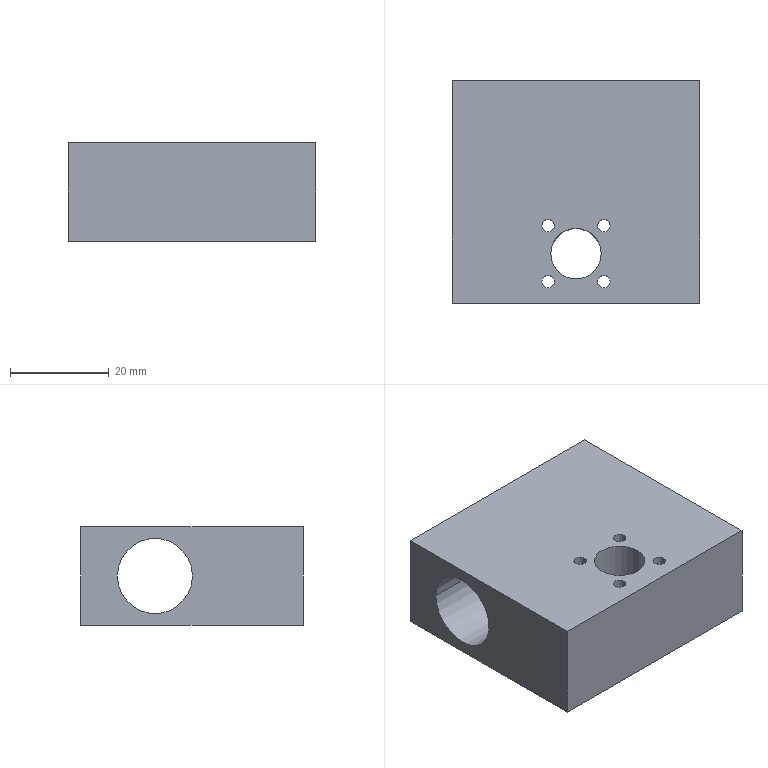Component | SolidWorks | Slider-1 | 1 solid | 18 faces | box 50 x 45 x 20 mm | volume 33900 mm3 | cylinder 12 | plane 6 | commonest cylinder face diameters 2.5 x8 15.2 x2 10.2 x2
STEP:
#1=CARTESIAN_POINT('',(0.9843,1.087,3.119));
#2=VERTEX_POINT('',#1);
#3=CARTESIAN_POINT('',(0.9843,0.4882,3.119));
#4=VERTEX_POINT('',#3);
#5=CARTESIAN_POINT('',(0.9843,0.7874,3.119));
#6=DIRECTION('',(-1.,-0.,0.));
#7=DIRECTION('',(-0.,1.,0.));
#8=AXIS2_PLACEMENT_3D('',#5,#6,#7);
#9=CIRCLE('',#8,0.2992);
#10=EDGE_CURVE('',#2,#4,#9,.T.);
#11=ORIENTED_EDGE('',*,*,#10,.F.);
#12=CARTESIAN_POINT('',(-0.9843,1.087,3.119));
#13=VERTEX_POINT('',#12);
#14=CARTESIAN_POINT('',(1.831,1.087,3.119));
#15=DIRECTION('',(-1.,-0.,0.));
#16=VECTOR('',#15,39.37);
#17=LINE('',#14,#16);
#18=EDGE_CURVE('',#2,#13,#17,.T.);
#19=ORIENTED_EDGE('',*,*,#18,.T.);
#20=CARTESIAN_POINT('',(-0.9843,0.4882,3.119));
#21=VERTEX_POINT('',#20);
#22=CARTESIAN_POINT('',(-0.9843,0.7874,3.119));
#23=DIRECTION('',(-1.,-0.,0.));
#24=DIRECTION('',(0.,-1.,0.));
#25=AXIS2_PLACEMENT_3D('',#22,#23,#24);
#26=CIRCLE('',#25,0.2992);
#27=EDGE_CURVE('',#13,#21,#26,.T.);
#28=ORIENTED_EDGE('',*,*,#27,.T.);
#29=CARTESIAN_POINT('',(1.831,0.4882,3.119));
#30=DIRECTION('',(-1.,-0.,0.));
#31=VECTOR('',#30,39.37);
#32=LINE('',#29,#31);
#33=EDGE_CURVE('',#4,#21,#32,.T.);
#34=ORIENTED_EDGE('',*,*,#33,.F.);
#35=EDGE_LOOP('',(#11,#19,#28,#34));
#36=FACE_OUTER_BOUND('',#35,.T.);
#37=CARTESIAN_POINT('',(1.831,0.7874,3.119));
#38=DIRECTION('',(-1.,-0.,0.));
#39=DIRECTION('',(0.,-1.,0.));
#40=AXIS2_PLACEMENT_3D('',#37,#38,#39);
#41=CYLINDRICAL_SURFACE('',#40,0.2992);
#42=ADVANCED_FACE('',(#36),#41,.F.);
#43=CARTESIAN_POINT('',(0.2719,-0.2227,2.725));
#44=VERTEX_POINT('',#43);
#45=CARTESIAN_POINT('',(0.1735,-0.2227,2.725));
#46=VERTEX_POINT('',#45);
#47=CARTESIAN_POINT('',(0.2227,-0.2227,2.725));
#48=DIRECTION('',(0.,0.,-1.));
#49=DIRECTION('',(1.,0.,0.));
#50=AXIS2_PLACEMENT_3D('',#47,#48,#49);
#51=CIRCLE('',#50,0.04921);
#52=EDGE_CURVE('',#44,#46,#51,.T.);
#53=ORIENTED_EDGE('',*,*,#52,.T.);
#54=CARTESIAN_POINT('',(0.1735,-0.2227,3.512));
#55=VERTEX_POINT('',#54);
#56=CARTESIAN_POINT('',(0.1735,-0.2227,2.586));
#57=DIRECTION('',(0.,0.,1.));
#58=VECTOR('',#57,39.37);
#59=LINE('',#56,#58);
#60=EDGE_CURVE('',#46,#55,#59,.T.);
#61=ORIENTED_EDGE('',*,*,#60,.T.);
#62=CARTESIAN_POINT('',(0.2719,-0.2227,3.512));
#63=VERTEX_POINT('',#62);
#64=CARTESIAN_POINT('',(0.2227,-0.2227,3.512));
#65=DIRECTION('',(0.,0.,1.));
#66=DIRECTION('',(1.,0.,0.));
#67=AXIS2_PLACEMENT_3D('',#64,#65,#66);
#68=CIRCLE('',#67,0.04921);
#69=EDGE_CURVE('',#55,#63,#68,.T.);
#70=ORIENTED_EDGE('',*,*,#69,.T.);
#71=CARTESIAN_POINT('',(0.2719,-0.2227,2.586));
#72=DIRECTION('',(0.,0.,1.));
#73=VECTOR('',#72,39.37);
#74=LINE('',#71,#73);
#75=EDGE_CURVE('',#44,#63,#74,.T.);
#76=ORIENTED_EDGE('',*,*,#75,.F.);
#77=EDGE_LOOP('',(#53,#61,#70,#76));
#78=FACE_OUTER_BOUND('',#77,.T.);
#79=CARTESIAN_POINT('',(0.2227,-0.2227,2.586));
#80=DIRECTION('',(0.,0.,1.));
#81=DIRECTION('',(1.,0.,0.));
#82=AXIS2_PLACEMENT_3D('',#79,#80,#81);
#83=CYLINDRICAL_SURFACE('',#82,0.04921);
#84=ADVANCED_FACE('',(#78),#83,.F.);
#85=CARTESIAN_POINT('',(-0.1735,-0.2227,2.725));
#86=VERTEX_POINT('',#85);
#87=CARTESIAN_POINT('',(-0.2719,-0.2227,2.725));
#88=VERTEX_POINT('',#87);
#89=CARTESIAN_POINT('',(-0.2227,-0.2227,2.725));
#90=DIRECTION('',(0.,0.,-1.));
#91=DIRECTION('',(1.,0.,0.));
#92=AXIS2_PLACEMENT_3D('',#89,#90,#91);
#93=CIRCLE('',#92,0.04921);
#94=EDGE_CURVE('',#86,#88,#93,.T.);
#95=ORIENTED_EDGE('',*,*,#94,.T.);
#96=CARTESIAN_POINT('',(-0.2719,-0.2227,3.512));
#97=VERTEX_POINT('',#96);
#98=CARTESIAN_POINT('',(-0.2719,-0.2227,2.586));
#99=DIRECTION('',(0.,0.,1.));
#100=VECTOR('',#99,39.37);
#101=LINE('',#98,#100);
#102=EDGE_CURVE('',#88,#97,#101,.T.);
#103=ORIENTED_EDGE('',*,*,#102,.T.);
#104=CARTESIAN_POINT('',(-0.1735,-0.2227,3.512));
#105=VERTEX_POINT('',#104);
#106=CARTESIAN_POINT('',(-0.2227,-0.2227,3.512));
#107=DIRECTION('',(0.,0.,1.));
#108=DIRECTION('',(1.,0.,0.));
#109=AXIS2_PLACEMENT_3D('',#106,#107,#108);
#110=CIRCLE('',#109,0.04921);
#111=EDGE_CURVE('',#97,#105,#110,.T.);
#112=ORIENTED_EDGE('',*,*,#111,.T.);
#113=CARTESIAN_POINT('',(-0.1735,-0.2227,2.586));
#114=DIRECTION('',(0.,0.,1.));
#115=VECTOR('',#114,39.37);
#116=LINE('',#113,#115);
#117=EDGE_CURVE('',#86,#105,#116,.T.);
#118=ORIENTED_EDGE('',*,*,#117,.F.);
#119=EDGE_LOOP('',(#95,#103,#112,#118));
#120=FACE_OUTER_BOUND('',#119,.T.);
#121=CARTESIAN_POINT('',(-0.2227,-0.2227,2.586));
#122=DIRECTION('',(0.,0.,1.));
#123=DIRECTION('',(1.,0.,0.));
#124=AXIS2_PLACEMENT_3D('',#121,#122,#123);
#125=CYLINDRICAL_SURFACE('',#124,0.04921);
#126=ADVANCED_FACE('',(#120),#125,.F.);
#127=CARTESIAN_POINT('',(0.2719,0.2227,2.725));
#128=VERTEX_POINT('',#127);
#129=CARTESIAN_POINT('',(0.1735,0.2227,2.725));
#130=VERTEX_POINT('',#129);
#131=CARTESIAN_POINT('',(0.2227,0.2227,2.725));
#132=DIRECTION('',(0.,0.,-1.));
#133=DIRECTION('',(1.,0.,0.));
#134=AXIS2_PLACEMENT_3D('',#131,#132,#133);
#135=CIRCLE('',#134,0.04921);
#136=EDGE_CURVE('',#128,#130,#135,.T.);
#137=ORIENTED_EDGE('',*,*,#136,.T.);
#138=CARTESIAN_POINT('',(0.1735,0.2227,3.512));
#139=VERTEX_POINT('',#138);
#140=CARTESIAN_POINT('',(0.1735,0.2227,2.586));
#141=DIRECTION('',(0.,0.,1.));
#142=VECTOR('',#141,39.37);
#143=LINE('',#140,#142);
#144=EDGE_CURVE('',#130,#139,#143,.T.);
#145=ORIENTED_EDGE('',*,*,#144,.T.);
#146=CARTESIAN_POINT('',(0.2719,0.2227,3.512));
#147=VERTEX_POINT('',#146);
#148=CARTESIAN_POINT('',(0.2227,0.2227,3.512));
#149=DIRECTION('',(0.,0.,1.));
#150=DIRECTION('',(1.,0.,0.));
#151=AXIS2_PLACEMENT_3D('',#148,#149,#150);
#152=CIRCLE('',#151,0.04921);
#153=EDGE_CURVE('',#139,#147,#152,.T.);
#154=ORIENTED_EDGE('',*,*,#153,.T.);
#155=CARTESIAN_POINT('',(0.2719,0.2227,2.586));
#156=DIRECTION('',(0.,0.,1.));
#157=VECTOR('',#156,39.37);
#158=LINE('',#155,#157);
#159=EDGE_CURVE('',#128,#147,#158,.T.);
#160=ORIENTED_EDGE('',*,*,#159,.F.);
#161=EDGE_LOOP('',(#137,#145,#154,#160));
#162=FACE_OUTER_BOUND('',#161,.T.);
#163=CARTESIAN_POINT('',(0.2227,0.2227,2.586));
#164=DIRECTION('',(0.,0.,1.));
#165=DIRECTION('',(1.,0.,0.));
#166=AXIS2_PLACEMENT_3D('',#163,#164,#165);
#167=CYLINDRICAL_SURFACE('',#166,0.04921);
#168=ADVANCED_FACE('',(#162),#167,.F.);
#169=CARTESIAN_POINT('',(-0.1735,0.2227,2.725));
#170=VERTEX_POINT('',#169);
#171=CARTESIAN_POINT('',(-0.2719,0.2227,2.725));
#172=VERTEX_POINT('',#171);
#173=CARTESIAN_POINT('',(-0.2227,0.2227,2.725));
#174=DIRECTION('',(0.,0.,-1.));
#175=DIRECTION('',(1.,0.,0.));
#176=AXIS2_PLACEMENT_3D('',#173,#174,#175);
#177=CIRCLE('',#176,0.04921);
#178=EDGE_CURVE('',#170,#172,#177,.T.);
#179=ORIENTED_EDGE('',*,*,#178,.T.);
#180=CARTESIAN_POINT('',(-0.2719,0.2227,3.512));
#181=VERTEX_POINT('',#180);
#182=CARTESIAN_POINT('',(-0.2719,0.2227,2.586));
#183=DIRECTION('',(0.,0.,1.));
#184=VECTOR('',#183,39.37);
#185=LINE('',#182,#184);
#186=EDGE_CURVE('',#172,#181,#185,.T.);
#187=ORIENTED_EDGE('',*,*,#186,.T.);
#188=CARTESIAN_POINT('',(-0.1735,0.2227,3.512));
#189=VERTEX_POINT('',#188);
#190=CARTESIAN_POINT('',(-0.2227,0.2227,3.512));
#191=DIRECTION('',(0.,0.,1.));
#192=DIRECTION('',(1.,0.,0.));
#193=AXIS2_PLACEMENT_3D('',#190,#191,#192);
#194=CIRCLE('',#193,0.04921);
#195=EDGE_CURVE('',#181,#189,#194,.T.);
#196=ORIENTED_EDGE('',*,*,#195,.T.);
#197=CARTESIAN_POINT('',(-0.1735,0.2227,2.586));
#198=DIRECTION('',(0.,0.,1.));
#199=VECTOR('',#198,39.37);
#200=LINE('',#197,#199);
#201=EDGE_CURVE('',#170,#189,#200,.T.);
#202=ORIENTED_EDGE('',*,*,#201,.F.);
#203=EDGE_LOOP('',(#179,#187,#196,#202));
#204=FACE_OUTER_BOUND('',#203,.T.);
#205=CARTESIAN_POINT('',(-0.2227,0.2227,2.586));
#206=DIRECTION('',(0.,0.,1.));
#207=DIRECTION('',(1.,0.,0.));
#208=AXIS2_PLACEMENT_3D('',#205,#206,#207);
#209=CYLINDRICAL_SURFACE('',#208,0.04921);
#210=ADVANCED_FACE('',(#204),#209,.F.);
#211=CARTESIAN_POINT('',(0.2008,0.,2.725));
#212=VERTEX_POINT('',#211);
#213=CARTESIAN_POINT('',(-0.2008,0.,2.725));
#214=VERTEX_POINT('',#213);
#215=CARTESIAN_POINT('',(-0.,0.,2.725));
#216=DIRECTION('',(0.,0.,-1.));
#217=DIRECTION('',(1.,0.,0.));
#218=AXIS2_PLACEMENT_3D('',#215,#216,#217);
#219=CIRCLE('',#218,0.2008);
#220=EDGE_CURVE('',#212,#214,#219,.T.);
#221=ORIENTED_EDGE('',*,*,#220,.T.);
#222=CARTESIAN_POINT('',(-0.2008,0.,3.512));
#223=VERTEX_POINT('',#222);
#224=CARTESIAN_POINT('',(-0.2008,0.,2.157));
#225=DIRECTION('',(0.,0.,1.));
#226=VECTOR('',#225,39.37);
#227=LINE('',#224,#226);
#228=EDGE_CURVE('',#214,#223,#227,.T.);
#229=ORIENTED_EDGE('',*,*,#228,.T.);
#230=CARTESIAN_POINT('',(0.2008,0.,3.512));
#231=VERTEX_POINT('',#230);
#232=CARTESIAN_POINT('',(-0.,0.,3.512));
#233=DIRECTION('',(0.,0.,1.));
#234=DIRECTION('',(1.,0.,0.));
#235=AXIS2_PLACEMENT_3D('',#232,#233,#234);
#236=CIRCLE('',#235,0.2008);
#237=EDGE_CURVE('',#223,#231,#236,.T.);
#238=ORIENTED_EDGE('',*,*,#237,.T.);
#239=CARTESIAN_POINT('',(0.2008,0.,2.157));
#240=DIRECTION('',(0.,0.,1.));
#241=VECTOR('',#240,39.37);
#242=LINE('',#239,#241);
#243=EDGE_CURVE('',#212,#231,#242,.T.);
#244=ORIENTED_EDGE('',*,*,#243,.F.);
#245=EDGE_LOOP('',(#221,#229,#238,#244));
#246=FACE_OUTER_BOUND('',#245,.T.);
#247=CARTESIAN_POINT('',(-0.,0.,2.157));
#248=DIRECTION('',(0.,0.,1.));
#249=DIRECTION('',(1.,0.,0.));
#250=AXIS2_PLACEMENT_3D('',#247,#248,#249);
#251=CYLINDRICAL_SURFACE('',#250,0.2008);
#252=ADVANCED_FACE('',(#246),#251,.F.);
#253=CARTESIAN_POINT('',(-0.9843,0.7874,3.119));
#254=DIRECTION('',(-1.,-0.,0.));
#255=DIRECTION('',(0.,-1.,0.));
#256=AXIS2_PLACEMENT_3D('',#253,#254,#255);
#257=CIRCLE('',#256,0.2992);
#258=EDGE_CURVE('',#21,#13,#257,.T.);
#259=ORIENTED_EDGE('',*,*,#258,.F.);
#260=ORIENTED_EDGE('',*,*,#27,.F.);
#261=EDGE_LOOP('',(#259,#260));
#262=FACE_BOUND('',#261,.T.);
#263=CARTESIAN_POINT('',(-0.9843,1.378,3.512));
#264=VERTEX_POINT('',#263);
#265=CARTESIAN_POINT('',(-0.9843,-0.3937,3.512));
#266=VERTEX_POINT('',#265);
#267=CARTESIAN_POINT('',(-0.9843,1.378,3.512));
#268=DIRECTION('',(0.,-1.,0.));
#269=VECTOR('',#268,39.37);
#270=LINE('',#267,#269);
#271=EDGE_CURVE('',#264,#266,#270,.T.);
#272=ORIENTED_EDGE('',*,*,#271,.F.);
#273=CARTESIAN_POINT('',(-0.9843,1.378,2.725));
#274=VERTEX_POINT('',#273);
#275=CARTESIAN_POINT('',(-0.9843,1.378,2.725));
#276=DIRECTION('',(0.,0.,1.));
#277=VECTOR('',#276,39.37);
#278=LINE('',#275,#277);
#279=EDGE_CURVE('',#274,#264,#278,.T.);
#280=ORIENTED_EDGE('',*,*,#279,.F.);
#281=CARTESIAN_POINT('',(-0.9843,-0.3937,2.725));
#282=VERTEX_POINT('',#281);
#283=CARTESIAN_POINT('',(-0.9843,1.378,2.725));
#284=DIRECTION('',(0.,-1.,0.));
#285=VECTOR('',#284,39.37);
#286=LINE('',#283,#285);
#287=EDGE_CURVE('',#274,#282,#286,.T.);
#288=ORIENTED_EDGE('',*,*,#287,.T.);
#289=CARTESIAN_POINT('',(-0.9843,-0.3937,2.725));
#290=DIRECTION('',(0.,0.,1.));
#291=VECTOR('',#290,39.37);
#292=LINE('',#289,#291);
#293=EDGE_CURVE('',#282,#266,#292,.T.);
#294=ORIENTED_EDGE('',*,*,#293,.T.);
#295=EDGE_LOOP('',(#272,#280,#288,#294));
#296=FACE_OUTER_BOUND('',#295,.T.);
#297=CARTESIAN_POINT('',(-0.9843,1.378,2.725));
#298=DIRECTION('',(-1.,-0.,0.));
#299=DIRECTION('',(0.,-1.,0.));
#300=AXIS2_PLACEMENT_3D('',#297,#298,#299);
#301=PLANE('',#300);
#302=ADVANCED_FACE('',(#262,#296),#301,.T.);
#303=CARTESIAN_POINT('',(0.9843,1.378,3.512));
#304=VERTEX_POINT('',#303);
#305=CARTESIAN_POINT('',(-0.9843,1.378,3.512));
#306=DIRECTION('',(-1.,-0.,0.));
#307=VECTOR('',#306,39.37);
#308=LINE('',#305,#307);
#309=EDGE_CURVE('',#304,#264,#308,.T.);
#310=ORIENTED_EDGE('',*,*,#309,.F.);
#311=CARTESIAN_POINT('',(0.9843,1.378,2.725));
#312=VERTEX_POINT('',#311);
#313=CARTESIAN_POINT('',(0.9843,1.378,2.725));
#314=DIRECTION('',(0.,0.,1.));
#315=VECTOR('',#314,39.37);
#316=LINE('',#313,#315);
#317=EDGE_CURVE('',#312,#304,#316,.T.);
#318=ORIENTED_EDGE('',*,*,#317,.F.);
#319=CARTESIAN_POINT('',(-0.9843,1.378,2.725));
#320=DIRECTION('',(-1.,-0.,0.));
#321=VECTOR('',#320,39.37);
#322=LINE('',#319,#321);
#323=EDGE_CURVE('',#312,#274,#322,.T.);
#324=ORIENTED_EDGE('',*,*,#323,.T.);
#325=ORIENTED_EDGE('',*,*,#279,.T.);
#326=EDGE_LOOP('',(#310,#318,#324,#325));
#327=FACE_OUTER_BOUND('',#326,.T.);
#328=CARTESIAN_POINT('',(-0.9843,1.378,2.725));
#329=DIRECTION('',(-0.,1.,0.));
#330=DIRECTION('',(-1.,-0.,0.));
#331=AXIS2_PLACEMENT_3D('',#328,#329,#330);
#332=PLANE('',#331);
#333=ADVANCED_FACE('',(#327),#332,.T.);
#334=CARTESIAN_POINT('',(0.9843,0.7874,3.119));
#335=DIRECTION('',(-1.,-0.,0.));
#336=DIRECTION('',(-0.,1.,0.));
#337=AXIS2_PLACEMENT_3D('',#334,#335,#336);
#338=CIRCLE('',#337,0.2992);
#339=EDGE_CURVE('',#4,#2,#338,.T.);
#340=ORIENTED_EDGE('',*,*,#339,.T.);
#341=ORIENTED_EDGE('',*,*,#10,.T.);
#342=EDGE_LOOP('',(#340,#341));
#343=FACE_BOUND('',#342,.T.);
#344=CARTESIAN_POINT('',(0.9843,-0.3937,3.512));
#345=VERTEX_POINT('',#344);
#346=CARTESIAN_POINT('',(0.9843,1.378,3.512));
#347=DIRECTION('',(-0.,1.,0.));
#348=VECTOR('',#347,39.37);
#349=LINE('',#346,#348);
#350=EDGE_CURVE('',#345,#304,#349,.T.);
#351=ORIENTED_EDGE('',*,*,#350,.F.);
#352=CARTESIAN_POINT('',(0.9843,-0.3937,2.725));
#353=VERTEX_POINT('',#352);
#354=CARTESIAN_POINT('',(0.9843,-0.3937,2.725));
#355=DIRECTION('',(0.,0.,1.));
#356=VECTOR('',#355,39.37);
#357=LINE('',#354,#356);
#358=EDGE_CURVE('',#353,#345,#357,.T.);
#359=ORIENTED_EDGE('',*,*,#358,.F.);
#360=CARTESIAN_POINT('',(0.9843,1.378,2.725));
#361=DIRECTION('',(-0.,1.,0.));
#362=VECTOR('',#361,39.37);
#363=LINE('',#360,#362);
#364=EDGE_CURVE('',#353,#312,#363,.T.);
#365=ORIENTED_EDGE('',*,*,#364,.T.);
#366=ORIENTED_EDGE('',*,*,#317,.T.);
#367=EDGE_LOOP('',(#351,#359,#365,#366));
#368=FACE_OUTER_BOUND('',#367,.T.);
#369=CARTESIAN_POINT('',(0.9843,1.378,2.725));
#370=DIRECTION('',(1.,0.,0.));
#371=DIRECTION('',(-0.,1.,0.));
#372=AXIS2_PLACEMENT_3D('',#369,#370,#371);
#373=PLANE('',#372);
#374=ADVANCED_FACE('',(#343,#368),#373,.T.);
#375=CARTESIAN_POINT('',(-0.9843,-0.3937,3.512));
#376=DIRECTION('',(1.,0.,0.));
#377=VECTOR('',#376,39.37);
#378=LINE('',#375,#377);
#379=EDGE_CURVE('',#266,#345,#378,.T.);
#380=ORIENTED_EDGE('',*,*,#379,.F.);
#381=ORIENTED_EDGE('',*,*,#293,.F.);
#382=CARTESIAN_POINT('',(-0.9843,-0.3937,2.725));
#383=DIRECTION('',(1.,0.,0.));
#384=VECTOR('',#383,39.37);
#385=LINE('',#382,#384);
#386=EDGE_CURVE('',#282,#353,#385,.T.);
#387=ORIENTED_EDGE('',*,*,#386,.T.);
#388=ORIENTED_EDGE('',*,*,#358,.T.);
#389=EDGE_LOOP('',(#380,#381,#387,#388));
#390=FACE_OUTER_BOUND('',#389,.T.);
#391=CARTESIAN_POINT('',(-0.9843,-0.3937,2.725));
#392=DIRECTION('',(0.,-1.,0.));
#393=DIRECTION('',(1.,0.,0.));
#394=AXIS2_PLACEMENT_3D('',#391,#392,#393);
#395=PLANE('',#394);
#396=ADVANCED_FACE('',(#390),#395,.T.);
#397=ORIENTED_EDGE('',*,*,#52,.F.);
#398=CARTESIAN_POINT('',(0.2227,-0.2227,2.725));
#399=DIRECTION('',(0.,0.,-1.));
#400=DIRECTION('',(1.,0.,0.));
#401=AXIS2_PLACEMENT_3D('',#398,#399,#400);
#402=CIRCLE('',#401,0.04921);
#403=EDGE_CURVE('',#46,#44,#402,.T.);
#404=ORIENTED_EDGE('',*,*,#403,.F.);
#405=EDGE_LOOP('',(#397,#404));
#406=FACE_BOUND('',#405,.T.);
#407=ORIENTED_EDGE('',*,*,#94,.F.);
#408=CARTESIAN_POINT('',(-0.2227,-0.2227,2.725));
#409=DIRECTION('',(0.,0.,-1.));
#410=DIRECTION('',(1.,0.,0.));
#411=AXIS2_PLACEMENT_3D('',#408,#409,#410);
#412=CIRCLE('',#411,0.04921);
#413=EDGE_CURVE('',#88,#86,#412,.T.);
#414=ORIENTED_EDGE('',*,*,#413,.F.);
#415=EDGE_LOOP('',(#407,#414));
#416=FACE_BOUND('',#415,.T.);
#417=ORIENTED_EDGE('',*,*,#136,.F.);
#418=CARTESIAN_POINT('',(0.2227,0.2227,2.725));
#419=DIRECTION('',(0.,0.,-1.));
#420=DIRECTION('',(1.,0.,0.));
#421=AXIS2_PLACEMENT_3D('',#418,#419,#420);
#422=CIRCLE('',#421,0.04921);
#423=EDGE_CURVE('',#130,#128,#422,.T.);
#424=ORIENTED_EDGE('',*,*,#423,.F.);
#425=EDGE_LOOP('',(#417,#424));
#426=FACE_BOUND('',#425,.T.);
#427=ORIENTED_EDGE('',*,*,#178,.F.);
#428=CARTESIAN_POINT('',(-0.2227,0.2227,2.725));
#429=DIRECTION('',(0.,0.,-1.));
#430=DIRECTION('',(1.,0.,0.));
#431=AXIS2_PLACEMENT_3D('',#428,#429,#430);
#432=CIRCLE('',#431,0.04921);
#433=EDGE_CURVE('',#172,#170,#432,.T.);
#434=ORIENTED_EDGE('',*,*,#433,.F.);
#435=EDGE_LOOP('',(#427,#434));
#436=FACE_BOUND('',#435,.T.);
#437=ORIENTED_EDGE('',*,*,#220,.F.);
#438=CARTESIAN_POINT('',(-0.,0.,2.725));
#439=DIRECTION('',(0.,0.,-1.));
#440=DIRECTION('',(1.,0.,0.));
#441=AXIS2_PLACEMENT_3D('',#438,#439,#440);
#442=CIRCLE('',#441,0.2008);
#443=EDGE_CURVE('',#214,#212,#442,.T.);
#444=ORIENTED_EDGE('',*,*,#443,.F.);
#445=EDGE_LOOP('',(#437,#444));
#446=FACE_BOUND('',#445,.T.);
#447=ORIENTED_EDGE('',*,*,#287,.F.);
#448=ORIENTED_EDGE('',*,*,#323,.F.);
#449=ORIENTED_EDGE('',*,*,#364,.F.);
#450=ORIENTED_EDGE('',*,*,#386,.F.);
#451=EDGE_LOOP('',(#447,#448,#449,#450));
#452=FACE_OUTER_BOUND('',#451,.T.);
#453=CARTESIAN_POINT('',(-0.,0.4921,2.725));
#454=DIRECTION('',(0.,0.,1.));
#455=DIRECTION('',(1.,0.,0.));
#456=AXIS2_PLACEMENT_3D('',#453,#454,#455);
#457=PLANE('',#456);
#458=ADVANCED_FACE('',(#406,#416,#426,#436,#446,#452),#457,.F.);
#459=CARTESIAN_POINT('',(0.2227,-0.2227,3.512));
#460=DIRECTION('',(0.,0.,1.));
#461=DIRECTION('',(1.,0.,0.));
#462=AXIS2_PLACEMENT_3D('',#459,#460,#461);
#463=CIRCLE('',#462,0.04921);
#464=EDGE_CURVE('',#63,#55,#463,.T.);
#465=ORIENTED_EDGE('',*,*,#464,.F.);
#466=ORIENTED_EDGE('',*,*,#69,.F.);
#467=EDGE_LOOP('',(#465,#466));
#468=FACE_BOUND('',#467,.T.);
#469=CARTESIAN_POINT('',(-0.2227,-0.2227,3.512));
#470=DIRECTION('',(0.,0.,1.));
#471=DIRECTION('',(1.,0.,0.));
#472=AXIS2_PLACEMENT_3D('',#469,#470,#471);
#473=CIRCLE('',#472,0.04921);
#474=EDGE_CURVE('',#105,#97,#473,.T.);
#475=ORIENTED_EDGE('',*,*,#474,.F.);
#476=ORIENTED_EDGE('',*,*,#111,.F.);
#477=EDGE_LOOP('',(#475,#476));
#478=FACE_BOUND('',#477,.T.);
#479=CARTESIAN_POINT('',(0.2227,0.2227,3.512));
#480=DIRECTION('',(0.,0.,1.));
#481=DIRECTION('',(1.,0.,0.));
#482=AXIS2_PLACEMENT_3D('',#479,#480,#481);
#483=CIRCLE('',#482,0.04921);
#484=EDGE_CURVE('',#147,#139,#483,.T.);
#485=ORIENTED_EDGE('',*,*,#484,.F.);
#486=ORIENTED_EDGE('',*,*,#153,.F.);
#487=EDGE_LOOP('',(#485,#486));
#488=FACE_BOUND('',#487,.T.);
#489=CARTESIAN_POINT('',(-0.2227,0.2227,3.512));
#490=DIRECTION('',(0.,0.,1.));
#491=DIRECTION('',(1.,0.,0.));
#492=AXIS2_PLACEMENT_3D('',#489,#490,#491);
#493=CIRCLE('',#492,0.04921);
#494=EDGE_CURVE('',#189,#181,#493,.T.);
#495=ORIENTED_EDGE('',*,*,#494,.F.);
#496=ORIENTED_EDGE('',*,*,#195,.F.);
#497=EDGE_LOOP('',(#495,#496));
#498=FACE_BOUND('',#497,.T.);
#499=CARTESIAN_POINT('',(-0.,0.,3.512));
#500=DIRECTION('',(0.,0.,1.));
#501=DIRECTION('',(1.,0.,0.));
#502=AXIS2_PLACEMENT_3D('',#499,#500,#501);
#503=CIRCLE('',#502,0.2008);
#504=EDGE_CURVE('',#231,#223,#503,.T.);
#505=ORIENTED_EDGE('',*,*,#504,.F.);
#506=ORIENTED_EDGE('',*,*,#237,.F.);
#507=EDGE_LOOP('',(#505,#506));
#508=FACE_BOUND('',#507,.T.);
#509=ORIENTED_EDGE('',*,*,#271,.T.);
#510=ORIENTED_EDGE('',*,*,#379,.T.);
#511=ORIENTED_EDGE('',*,*,#350,.T.);
#512=ORIENTED_EDGE('',*,*,#309,.T.);
#513=EDGE_LOOP('',(#509,#510,#511,#512));
#514=FACE_OUTER_BOUND('',#513,.T.);
#515=CARTESIAN_POINT('',(-0.,0.4921,3.512));
#516=DIRECTION('',(0.,0.,1.));
#517=DIRECTION('',(1.,0.,0.));
#518=AXIS2_PLACEMENT_3D('',#515,#516,#517);
#519=PLANE('',#518);
#520=ADVANCED_FACE('',(#468,#478,#488,#498,#508,#514),#519,.T.);
#521=ORIENTED_EDGE('',*,*,#228,.F.);
#522=ORIENTED_EDGE('',*,*,#443,.T.);
#523=ORIENTED_EDGE('',*,*,#243,.T.);
#524=ORIENTED_EDGE('',*,*,#504,.T.);
#525=EDGE_LOOP('',(#521,#522,#523,#524));
#526=FACE_OUTER_BOUND('',#525,.T.);
#527=CARTESIAN_POINT('',(-0.,0.,2.157));
#528=DIRECTION('',(0.,0.,1.));
#529=DIRECTION('',(1.,0.,0.));
#530=AXIS2_PLACEMENT_3D('',#527,#528,#529);
#531=CYLINDRICAL_SURFACE('',#530,0.2008);
#532=ADVANCED_FACE('',(#526),#531,.F.);
#533=ORIENTED_EDGE('',*,*,#186,.F.);
#534=ORIENTED_EDGE('',*,*,#433,.T.);
#535=ORIENTED_EDGE('',*,*,#201,.T.);
#536=ORIENTED_EDGE('',*,*,#494,.T.);
#537=EDGE_LOOP('',(#533,#534,#535,#536));
#538=FACE_OUTER_BOUND('',#537,.T.);
#539=CARTESIAN_POINT('',(-0.2227,0.2227,2.586));
#540=DIRECTION('',(0.,0.,1.));
#541=DIRECTION('',(1.,0.,0.));
#542=AXIS2_PLACEMENT_3D('',#539,#540,#541);
#543=CYLINDRICAL_SURFACE('',#542,0.04921);
#544=ADVANCED_FACE('',(#538),#543,.F.);
#545=ORIENTED_EDGE('',*,*,#144,.F.);
#546=ORIENTED_EDGE('',*,*,#423,.T.);
#547=ORIENTED_EDGE('',*,*,#159,.T.);
#548=ORIENTED_EDGE('',*,*,#484,.T.);
#549=EDGE_LOOP('',(#545,#546,#547,#548));
#550=FACE_OUTER_BOUND('',#549,.T.);
#551=CARTESIAN_POINT('',(0.2227,0.2227,2.586));
#552=DIRECTION('',(0.,0.,1.));
#553=DIRECTION('',(1.,0.,0.));
#554=AXIS2_PLACEMENT_3D('',#551,#552,#553);
#555=CYLINDRICAL_SURFACE('',#554,0.04921);
#556=ADVANCED_FACE('',(#550),#555,.F.);
#557=ORIENTED_EDGE('',*,*,#102,.F.);
#558=ORIENTED_EDGE('',*,*,#413,.T.);
#559=ORIENTED_EDGE('',*,*,#117,.T.);
#560=ORIENTED_EDGE('',*,*,#474,.T.);
#561=EDGE_LOOP('',(#557,#558,#559,#560));
#562=FACE_OUTER_BOUND('',#561,.T.);
#563=CARTESIAN_POINT('',(-0.2227,-0.2227,2.586));
#564=DIRECTION('',(0.,0.,1.));
#565=DIRECTION('',(1.,0.,0.));
#566=AXIS2_PLACEMENT_3D('',#563,#564,#565);
#567=CYLINDRICAL_SURFACE('',#566,0.04921);
#568=ADVANCED_FACE('',(#562),#567,.F.);
#569=ORIENTED_EDGE('',*,*,#60,.F.);
#570=ORIENTED_EDGE('',*,*,#403,.T.);
#571=ORIENTED_EDGE('',*,*,#75,.T.);
#572=ORIENTED_EDGE('',*,*,#464,.T.);
#573=EDGE_LOOP('',(#569,#570,#571,#572));
#574=FACE_OUTER_BOUND('',#573,.T.);
#575=CARTESIAN_POINT('',(0.2227,-0.2227,2.586));
#576=DIRECTION('',(0.,0.,1.));
#577=DIRECTION('',(1.,0.,0.));
#578=AXIS2_PLACEMENT_3D('',#575,#576,#577);
#579=CYLINDRICAL_SURFACE('',#578,0.04921);
#580=ADVANCED_FACE('',(#574),#579,.F.);
#581=ORIENTED_EDGE('',*,*,#18,.F.);
#582=ORIENTED_EDGE('',*,*,#339,.F.);
#583=ORIENTED_EDGE('',*,*,#33,.T.);
#584=ORIENTED_EDGE('',*,*,#258,.T.);
#585=EDGE_LOOP('',(#581,#582,#583,#584));
#586=FACE_OUTER_BOUND('',#585,.T.);
#587=CARTESIAN_POINT('',(1.831,0.7874,3.119));
#588=DIRECTION('',(-1.,-0.,0.));
#589=DIRECTION('',(0.,-1.,0.));
#590=AXIS2_PLACEMENT_3D('',#587,#588,#589);
#591=CYLINDRICAL_SURFACE('',#590,0.2992);
#592=ADVANCED_FACE('',(#586),#591,.F.);
#593=CLOSED_SHELL('',(#42,#84,#126,#168,#210,#252,#302,#333,#374,#396,#458,#520,#532,#544,#556,#568,#580,#592));
#594=MANIFOLD_SOLID_BREP('',#593);
#595=CARTESIAN_POINT('',(0.,0.,0.));
#596=DIRECTION('',(0.,0.,1.));
#597=DIRECTION('',(1.,0.,0.));
#598=AXIS2_PLACEMENT_3D('',#595,#596,#597);
#599=(LENGTH_UNIT()NAMED_UNIT(*)SI_UNIT($,.METRE.));
#600=LENGTH_MEASURE_WITH_UNIT(LENGTH_MEASURE(0.0254),#599);
#601=DIMENSIONAL_EXPONENTS(1.,0.,0.,0.,0.,0.,0.);
#602=(CONVERSION_BASED_UNIT('',#600)LENGTH_UNIT()NAMED_UNIT(#601));
#603=UNCERTAINTY_MEASURE_WITH_UNIT(LENGTH_MEASURE(0.00001),#602,'','');
#604=(NAMED_UNIT(*)PLANE_ANGLE_UNIT()SI_UNIT($,.RADIAN.));
#605=(NAMED_UNIT(*)SI_UNIT($,.STERADIAN.)SOLID_ANGLE_UNIT());
#606=(GEOMETRIC_REPRESENTATION_CONTEXT(3)GLOBAL_UNCERTAINTY_ASSIGNED_CONTEXT((#603))GLOBAL_UNIT_ASSIGNED_CONTEXT((#602,#604,#605))REPRESENTATION_CONTEXT('',''));
#607=ADVANCED_BREP_SHAPE_REPRESENTATION('',(#594,#598),#606);
#608=COLOUR_RGB('',0.7922,0.8196,0.9333);
#609=FILL_AREA_STYLE_COLOUR('',#608);
#610=FILL_AREA_STYLE('',(#609));
#611=SURFACE_STYLE_FILL_AREA(#610);
#612=SURFACE_SIDE_STYLE('',(#611));
#613=SURFACE_STYLE_USAGE(.BOTH.,#612);
#614=PRESENTATION_STYLE_ASSIGNMENT((#613));
#615=STYLED_ITEM('',(#614),#594);
#616=PRESENTATION_LAYER_ASSIGNMENT('','',(#615));
#617=(LENGTH_UNIT()NAMED_UNIT(*)SI_UNIT($,.METRE.));
#618=LENGTH_MEASURE_WITH_UNIT(LENGTH_MEASURE(0.0254),#617);
#619=DIMENSIONAL_EXPONENTS(1.,0.,0.,0.,0.,0.,0.);
#620=(CONVERSION_BASED_UNIT('',#618)LENGTH_UNIT()NAMED_UNIT(#619));
#621=UNCERTAINTY_MEASURE_WITH_UNIT(LENGTH_MEASURE(0.00001),#620,'','');
#622=(NAMED_UNIT(*)PLANE_ANGLE_UNIT()SI_UNIT($,.RADIAN.));
#623=(NAMED_UNIT(*)SI_UNIT($,.STERADIAN.)SOLID_ANGLE_UNIT());
#624=(GEOMETRIC_REPRESENTATION_CONTEXT(3)GLOBAL_UNCERTAINTY_ASSIGNED_CONTEXT((#621))GLOBAL_UNIT_ASSIGNED_CONTEXT((#620,#622,#623))REPRESENTATION_CONTEXT('',''));
#625=MECHANICAL_DESIGN_GEOMETRIC_PRESENTATION_REPRESENTATION('',(#615),#624);